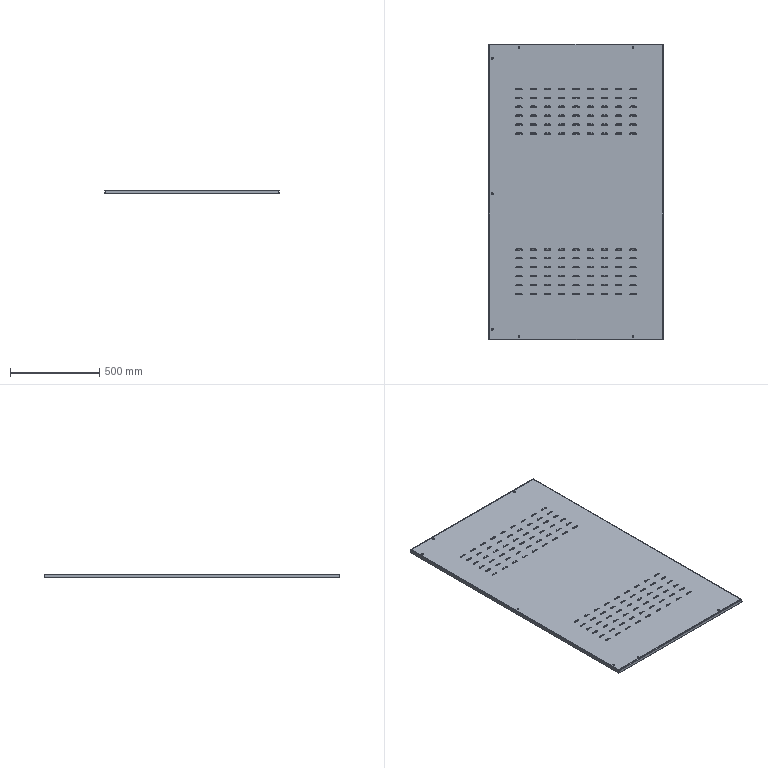Component | SolidWorks | SidePlate-2 | 1 solid | 1248 faces | volume 3437582 mm3 | sphere 432 | cylinder 346 | plane 246 | torus 216 | spline 8 | commonest cylinder face diameters 4 x112 12 x108 16 x108 10 x10 7 x4 8 x4